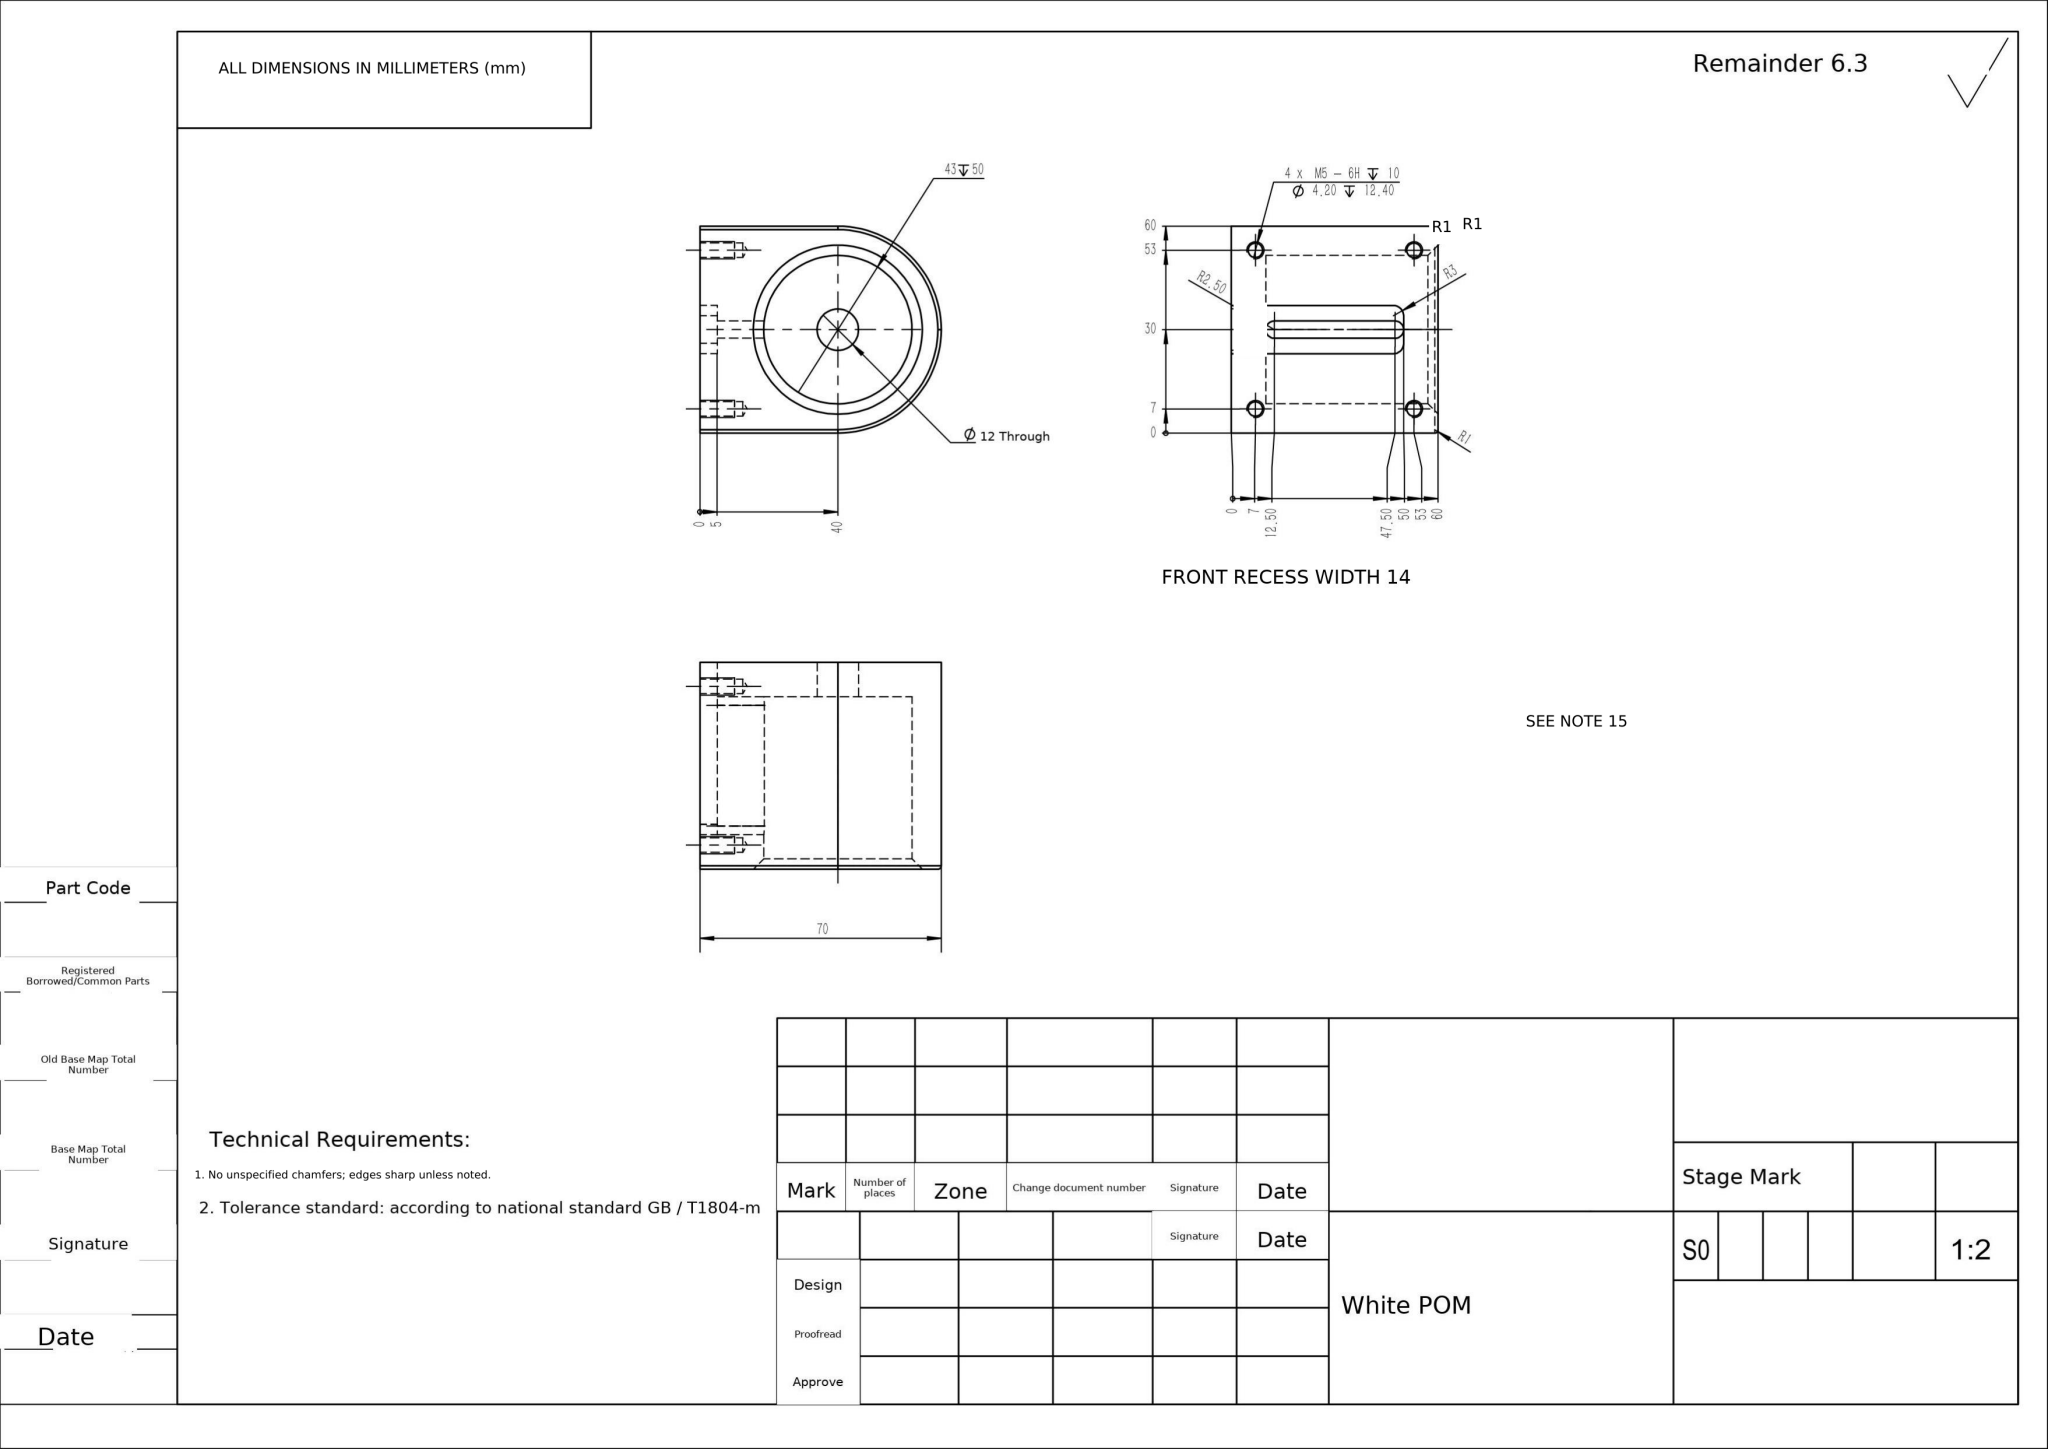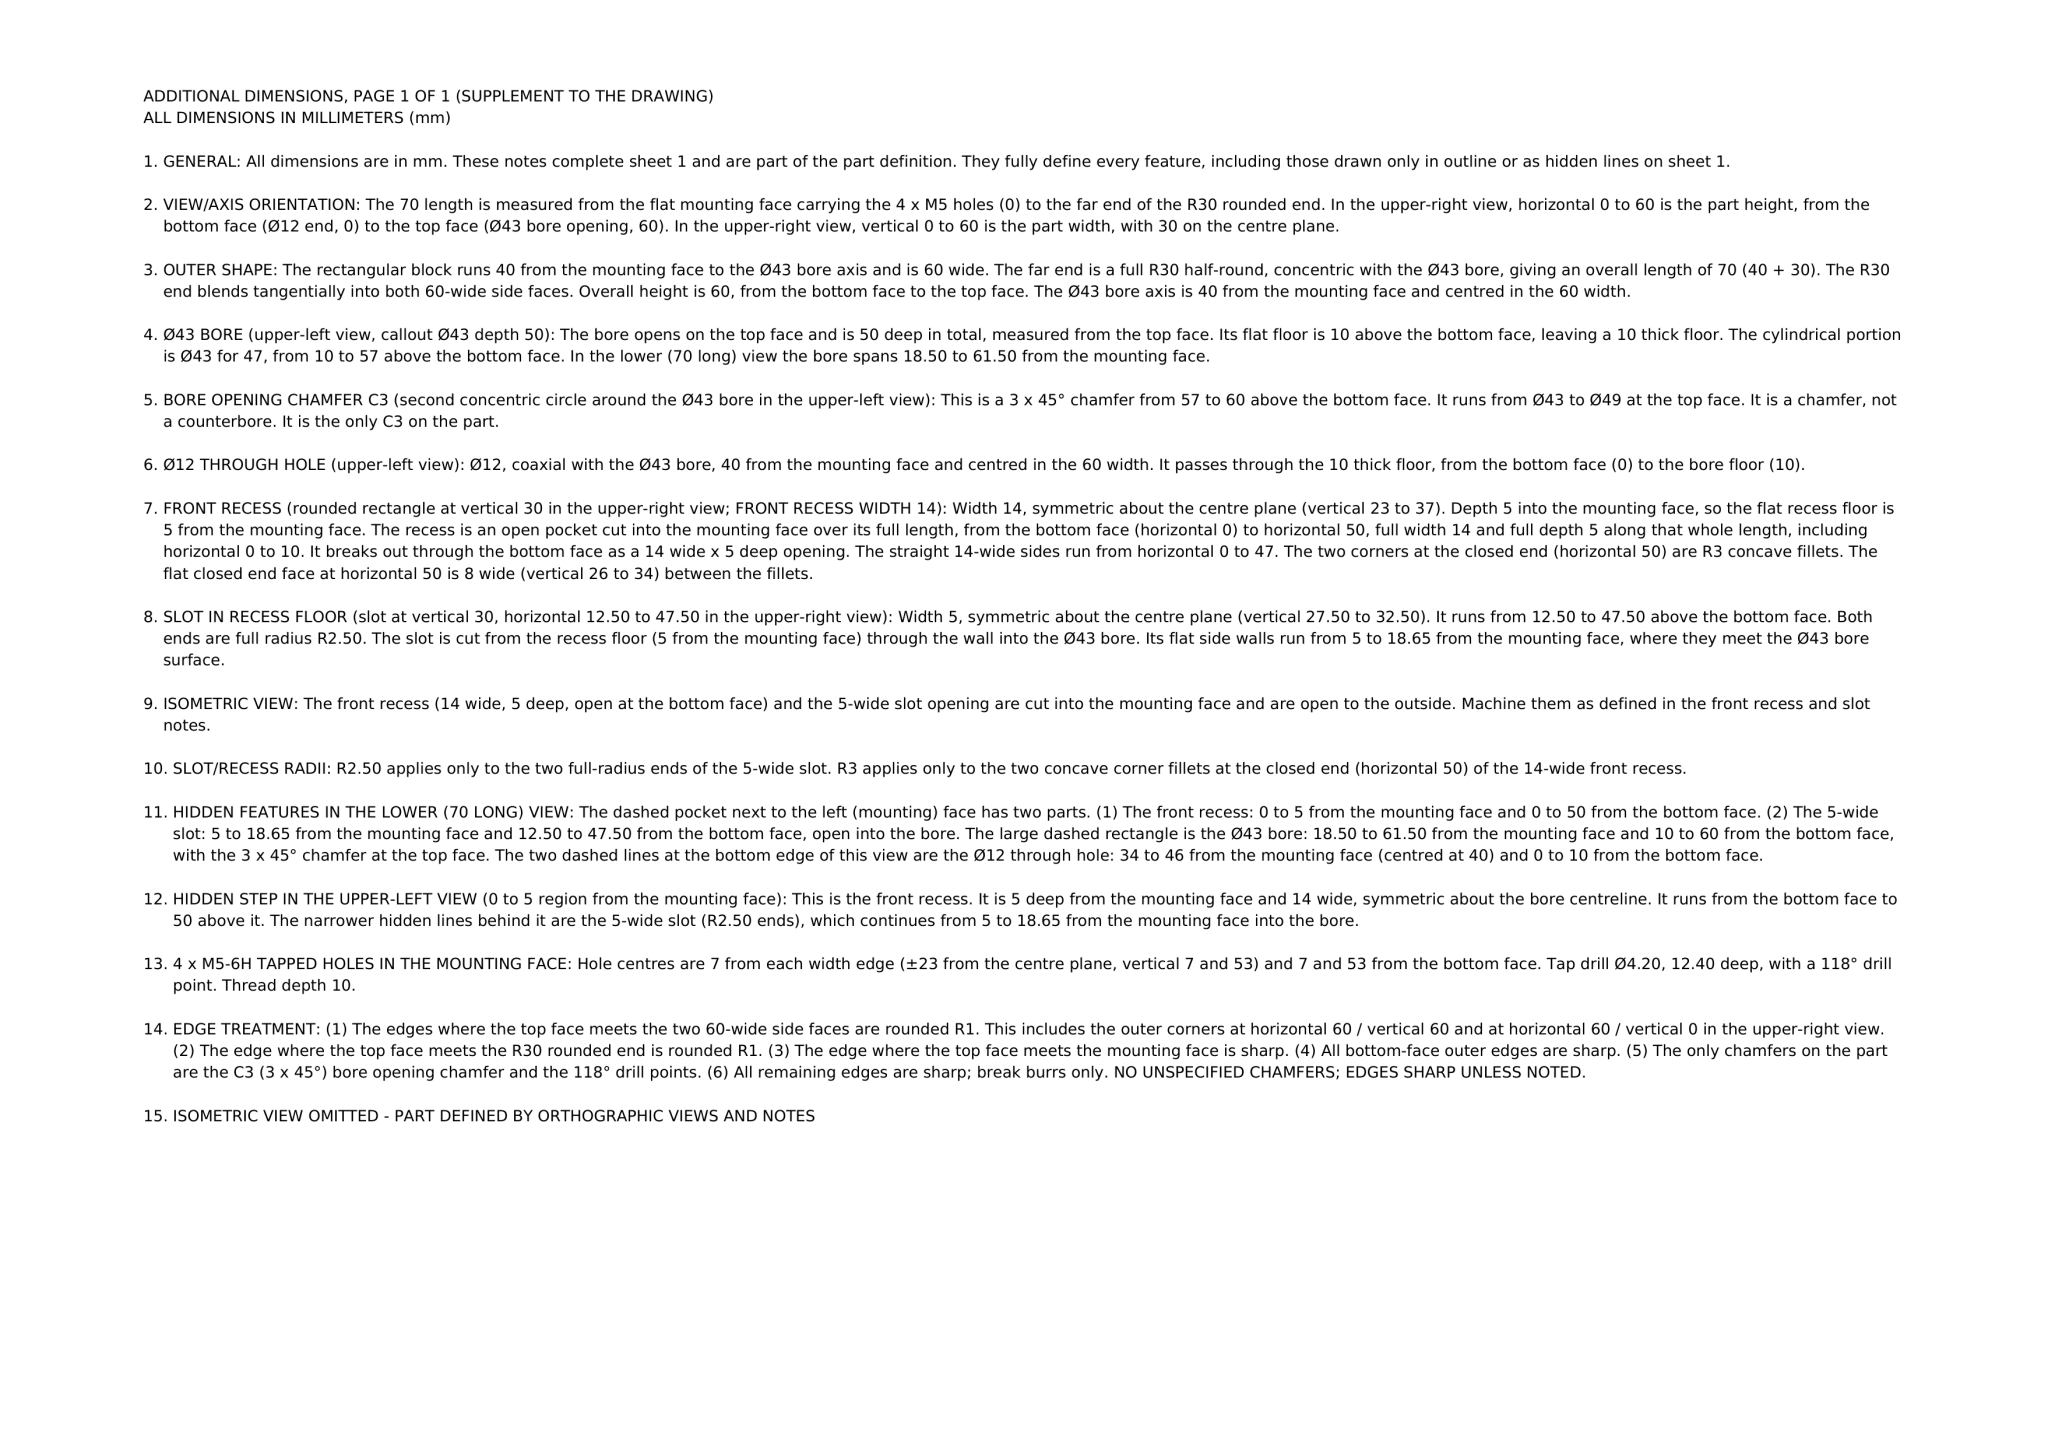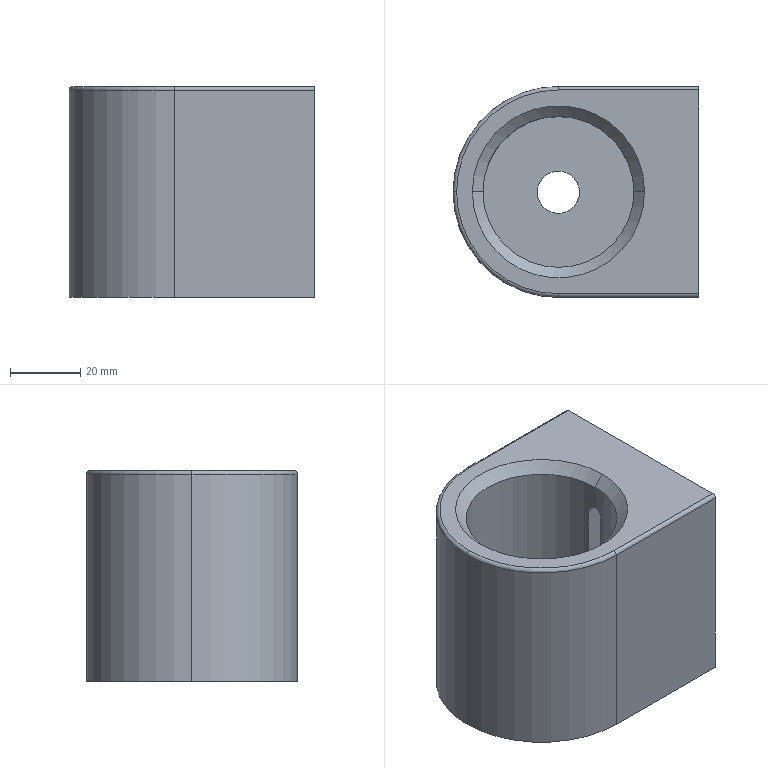Part | NX | mm | 1 solid | 45 faces | box 70 x 60 x 60 mm | volume 147581 mm3 | cylinder 21 | plane 12 | cone 10 | torus 2 | commonest cylinder face diameters 4.2 x8 5 x3 12 x2 43 x2 60 x2 6 x2 2 x2